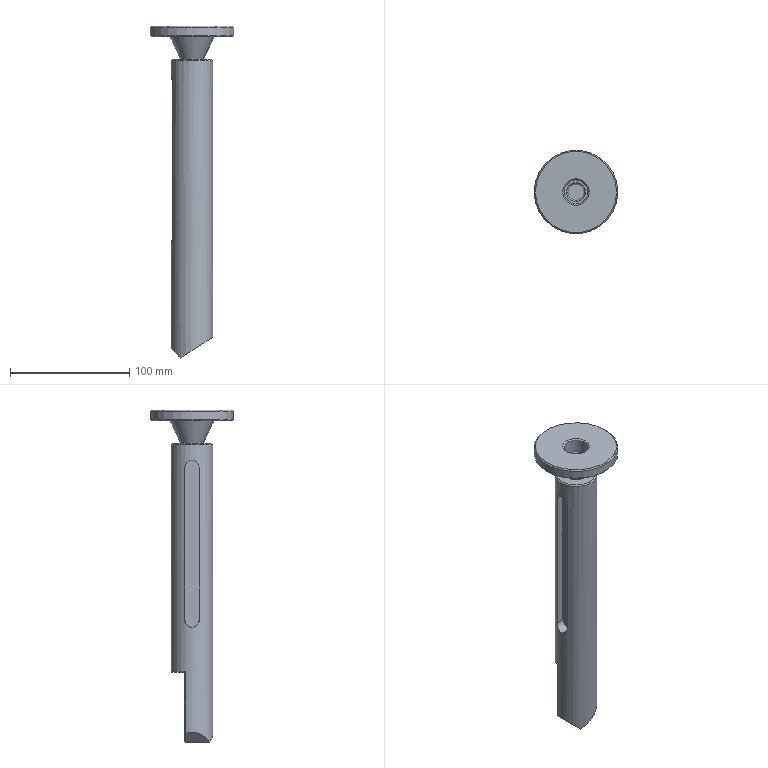Component | NX | YMSR_PET_P01 | 2 solids | 42 faces | volume 246187 mm3 | plane 16 | cone 15 | cylinder 10 | spline 1 | commonest cylinder face diameters 4.5 x4 12 x2 35 x1 70 x1 13.5 x1 20 x1